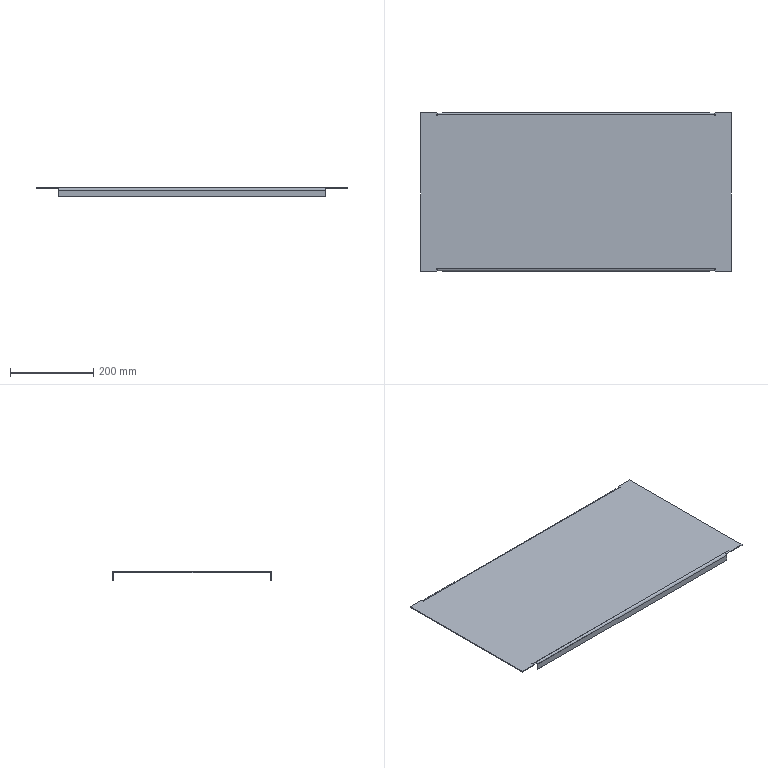Component | SolidWorks | Panel6-1 | 1 solid | 38 faces | volume 607029 mm3 | plane 34 | cylinder 4 | commonest cylinder face diameters 11 x2 7 x2 | material Malleable Cast Iron